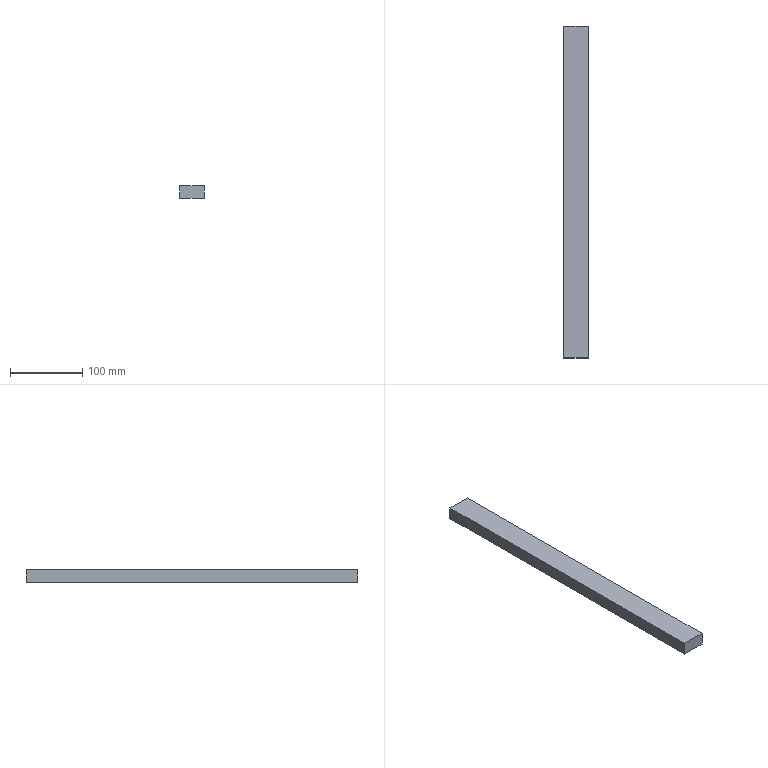Component | SolidWorks | SlideRailShim-3 | 1 solid | 6 faces | box 34 x 460 x 18 mm | volume 281520 mm3 | plane 6
build123d program:
from build123d import *

# Parameters (mm, degrees)
SKETCH1_W           = 18
SKETCH1_H           = 460
BOSS_EXTRUDE1_DEPTH = 17


with BuildPart() as part:
    # Sketch1 → Boss-Extrude1 (new, symmetric)
    with BuildSketch(Plane.XY):
        Rectangle(SKETCH1_W, SKETCH1_H)
    extrude(amount=BOSS_EXTRUDE1_DEPTH, both=True)


solid = part.part

# Placed as in the assembly
solid = solid.moved(Location((62.398, 237.837, 47.5), (0, 90, 0)))
STEP:
#1=CARTESIAN_POINT('',(3.126,18.419,1.516));
#2=VERTEX_POINT('',#1);
#3=CARTESIAN_POINT('',(3.126,0.3085,1.516));
#4=VERTEX_POINT('',#3);
#5=CARTESIAN_POINT('',(3.126,0.3085,1.516));
#6=DIRECTION('',(-0.,-1.,-0.));
#7=VECTOR('',#6,39.37);
#8=LINE('',#5,#7);
#9=EDGE_CURVE('',#2,#4,#8,.T.);
#10=ORIENTED_EDGE('',*,*,#9,.T.);
#11=CARTESIAN_POINT('',(1.787,0.3085,1.516));
#12=VERTEX_POINT('',#11);
#13=CARTESIAN_POINT('',(1.787,0.3085,1.516));
#14=DIRECTION('',(1.,0.,-0.));
#15=VECTOR('',#14,39.37);
#16=LINE('',#13,#15);
#17=EDGE_CURVE('',#12,#4,#16,.T.);
#18=ORIENTED_EDGE('',*,*,#17,.F.);
#19=CARTESIAN_POINT('',(1.787,18.419,1.516));
#20=VERTEX_POINT('',#19);
#21=CARTESIAN_POINT('',(1.787,0.3085,1.516));
#22=DIRECTION('',(-0.,-1.,-0.));
#23=VECTOR('',#22,39.37);
#24=LINE('',#21,#23);
#25=EDGE_CURVE('',#20,#12,#24,.T.);
#26=ORIENTED_EDGE('',*,*,#25,.F.);
#27=CARTESIAN_POINT('',(1.787,18.419,1.516));
#28=DIRECTION('',(1.,0.,-0.));
#29=VECTOR('',#28,39.37);
#30=LINE('',#27,#29);
#31=EDGE_CURVE('',#20,#2,#30,.T.);
#32=ORIENTED_EDGE('',*,*,#31,.T.);
#33=EDGE_LOOP('',(#10,#18,#26,#32));
#34=FACE_OUTER_BOUND('',#33,.T.);
#35=CARTESIAN_POINT('',(1.787,0.3085,1.516));
#36=DIRECTION('',(0.,-0.,1.));
#37=DIRECTION('',(1.,0.,-0.));
#38=AXIS2_PLACEMENT_3D('',#35,#36,#37);
#39=PLANE('',#38);
#40=ADVANCED_FACE('',(#34),#39,.F.);
#41=CARTESIAN_POINT('',(3.126,0.3085,2.224));
#42=VERTEX_POINT('',#41);
#43=CARTESIAN_POINT('',(3.126,0.3085,2.224));
#44=DIRECTION('',(0.,0.,1.));
#45=VECTOR('',#44,39.37);
#46=LINE('',#43,#45);
#47=EDGE_CURVE('',#4,#42,#46,.T.);
#48=ORIENTED_EDGE('',*,*,#47,.T.);
#49=CARTESIAN_POINT('',(1.787,0.3085,2.224));
#50=VERTEX_POINT('',#49);
#51=CARTESIAN_POINT('',(1.787,0.3085,2.224));
#52=DIRECTION('',(1.,0.,-0.));
#53=VECTOR('',#52,39.37);
#54=LINE('',#51,#53);
#55=EDGE_CURVE('',#50,#42,#54,.T.);
#56=ORIENTED_EDGE('',*,*,#55,.F.);
#57=CARTESIAN_POINT('',(1.787,0.3085,2.224));
#58=DIRECTION('',(0.,0.,1.));
#59=VECTOR('',#58,39.37);
#60=LINE('',#57,#59);
#61=EDGE_CURVE('',#12,#50,#60,.T.);
#62=ORIENTED_EDGE('',*,*,#61,.F.);
#63=ORIENTED_EDGE('',*,*,#17,.T.);
#64=EDGE_LOOP('',(#48,#56,#62,#63));
#65=FACE_OUTER_BOUND('',#64,.T.);
#66=CARTESIAN_POINT('',(1.787,0.3085,2.224));
#67=DIRECTION('',(-0.,1.,0.));
#68=DIRECTION('',(-1.,-0.,0.));
#69=AXIS2_PLACEMENT_3D('',#66,#67,#68);
#70=PLANE('',#69);
#71=ADVANCED_FACE('',(#65),#70,.F.);
#72=CARTESIAN_POINT('',(3.126,18.419,2.224));
#73=VERTEX_POINT('',#72);
#74=CARTESIAN_POINT('',(3.126,0.3085,2.224));
#75=DIRECTION('',(0.,1.,0.));
#76=VECTOR('',#75,39.37);
#77=LINE('',#74,#76);
#78=EDGE_CURVE('',#42,#73,#77,.T.);
#79=ORIENTED_EDGE('',*,*,#78,.T.);
#80=CARTESIAN_POINT('',(1.787,18.419,2.224));
#81=VERTEX_POINT('',#80);
#82=CARTESIAN_POINT('',(1.787,18.419,2.224));
#83=DIRECTION('',(1.,0.,-0.));
#84=VECTOR('',#83,39.37);
#85=LINE('',#82,#84);
#86=EDGE_CURVE('',#81,#73,#85,.T.);
#87=ORIENTED_EDGE('',*,*,#86,.F.);
#88=CARTESIAN_POINT('',(1.787,0.3085,2.224));
#89=DIRECTION('',(0.,1.,0.));
#90=VECTOR('',#89,39.37);
#91=LINE('',#88,#90);
#92=EDGE_CURVE('',#50,#81,#91,.T.);
#93=ORIENTED_EDGE('',*,*,#92,.F.);
#94=ORIENTED_EDGE('',*,*,#55,.T.);
#95=EDGE_LOOP('',(#79,#87,#93,#94));
#96=FACE_OUTER_BOUND('',#95,.T.);
#97=CARTESIAN_POINT('',(1.787,0.3085,2.224));
#98=DIRECTION('',(-0.,0.,-1.));
#99=DIRECTION('',(-1.,-0.,0.));
#100=AXIS2_PLACEMENT_3D('',#97,#98,#99);
#101=PLANE('',#100);
#102=ADVANCED_FACE('',(#96),#101,.F.);
#103=CARTESIAN_POINT('',(3.126,18.419,2.224));
#104=DIRECTION('',(-0.,0.,-1.));
#105=VECTOR('',#104,39.37);
#106=LINE('',#103,#105);
#107=EDGE_CURVE('',#73,#2,#106,.T.);
#108=ORIENTED_EDGE('',*,*,#107,.T.);
#109=ORIENTED_EDGE('',*,*,#31,.F.);
#110=CARTESIAN_POINT('',(1.787,18.419,2.224));
#111=DIRECTION('',(-0.,0.,-1.));
#112=VECTOR('',#111,39.37);
#113=LINE('',#110,#112);
#114=EDGE_CURVE('',#81,#20,#113,.T.);
#115=ORIENTED_EDGE('',*,*,#114,.F.);
#116=ORIENTED_EDGE('',*,*,#86,.T.);
#117=EDGE_LOOP('',(#108,#109,#115,#116));
#118=FACE_OUTER_BOUND('',#117,.T.);
#119=CARTESIAN_POINT('',(1.787,18.419,2.224));
#120=DIRECTION('',(0.,-1.,-0.));
#121=DIRECTION('',(1.,0.,-0.));
#122=AXIS2_PLACEMENT_3D('',#119,#120,#121);
#123=PLANE('',#122);
#124=ADVANCED_FACE('',(#118),#123,.F.);
#125=ORIENTED_EDGE('',*,*,#25,.T.);
#126=ORIENTED_EDGE('',*,*,#61,.T.);
#127=ORIENTED_EDGE('',*,*,#92,.T.);
#128=ORIENTED_EDGE('',*,*,#114,.T.);
#129=EDGE_LOOP('',(#125,#126,#127,#128));
#130=FACE_OUTER_BOUND('',#129,.T.);
#131=CARTESIAN_POINT('',(1.787,9.364,1.87));
#132=DIRECTION('',(-1.,-0.,0.));
#133=DIRECTION('',(0.,0.,1.));
#134=AXIS2_PLACEMENT_3D('',#131,#132,#133);
#135=PLANE('',#134);
#136=ADVANCED_FACE('',(#130),#135,.T.);
#137=ORIENTED_EDGE('',*,*,#9,.F.);
#138=ORIENTED_EDGE('',*,*,#107,.F.);
#139=ORIENTED_EDGE('',*,*,#78,.F.);
#140=ORIENTED_EDGE('',*,*,#47,.F.);
#141=EDGE_LOOP('',(#137,#138,#139,#140));
#142=FACE_OUTER_BOUND('',#141,.T.);
#143=CARTESIAN_POINT('',(3.126,9.364,1.87));
#144=DIRECTION('',(-1.,-0.,0.));
#145=DIRECTION('',(0.,0.,1.));
#146=AXIS2_PLACEMENT_3D('',#143,#144,#145);
#147=PLANE('',#146);
#148=ADVANCED_FACE('',(#142),#147,.F.);
#149=CLOSED_SHELL('',(#40,#71,#102,#124,#136,#148));
#150=MANIFOLD_SOLID_BREP('',#149);
#151=CARTESIAN_POINT('',(0.,0.,0.));
#152=DIRECTION('',(0.,0.,1.));
#153=DIRECTION('',(1.,0.,0.));
#154=AXIS2_PLACEMENT_3D('',#151,#152,#153);
#155=(LENGTH_UNIT()NAMED_UNIT(*)SI_UNIT($,.METRE.));
#156=LENGTH_MEASURE_WITH_UNIT(LENGTH_MEASURE(0.0254),#155);
#157=DIMENSIONAL_EXPONENTS(1.,0.,0.,0.,0.,0.,0.);
#158=(CONVERSION_BASED_UNIT('',#156)LENGTH_UNIT()NAMED_UNIT(#157));
#159=UNCERTAINTY_MEASURE_WITH_UNIT(LENGTH_MEASURE(0.00001),#158,'','');
#160=(NAMED_UNIT(*)PLANE_ANGLE_UNIT()SI_UNIT($,.RADIAN.));
#161=(NAMED_UNIT(*)SI_UNIT($,.STERADIAN.)SOLID_ANGLE_UNIT());
#162=(GEOMETRIC_REPRESENTATION_CONTEXT(3)GLOBAL_UNCERTAINTY_ASSIGNED_CONTEXT((#159))GLOBAL_UNIT_ASSIGNED_CONTEXT((#158,#160,#161))REPRESENTATION_CONTEXT('',''));
#163=ADVANCED_BREP_SHAPE_REPRESENTATION('',(#150,#154),#162);
#164=COLOUR_RGB('',0.7922,0.8196,0.9333);
#165=FILL_AREA_STYLE_COLOUR('',#164);
#166=FILL_AREA_STYLE('',(#165));
#167=SURFACE_STYLE_FILL_AREA(#166);
#168=SURFACE_SIDE_STYLE('',(#167));
#169=SURFACE_STYLE_USAGE(.BOTH.,#168);
#170=PRESENTATION_STYLE_ASSIGNMENT((#169));
#171=STYLED_ITEM('',(#170),#150);
#172=(LENGTH_UNIT()NAMED_UNIT(*)SI_UNIT($,.METRE.));
#173=LENGTH_MEASURE_WITH_UNIT(LENGTH_MEASURE(0.0254),#172);
#174=DIMENSIONAL_EXPONENTS(1.,0.,0.,0.,0.,0.,0.);
#175=(CONVERSION_BASED_UNIT('',#173)LENGTH_UNIT()NAMED_UNIT(#174));
#176=UNCERTAINTY_MEASURE_WITH_UNIT(LENGTH_MEASURE(0.00001),#175,'','');
#177=(NAMED_UNIT(*)PLANE_ANGLE_UNIT()SI_UNIT($,.RADIAN.));
#178=(NAMED_UNIT(*)SI_UNIT($,.STERADIAN.)SOLID_ANGLE_UNIT());
#179=(GEOMETRIC_REPRESENTATION_CONTEXT(3)GLOBAL_UNCERTAINTY_ASSIGNED_CONTEXT((#176))GLOBAL_UNIT_ASSIGNED_CONTEXT((#175,#177,#178))REPRESENTATION_CONTEXT('',''));
#180=MECHANICAL_DESIGN_GEOMETRIC_PRESENTATION_REPRESENTATION('',(#171),#179);
#181=PRESENTATION_LAYER_ASSIGNMENT('','',(#171));